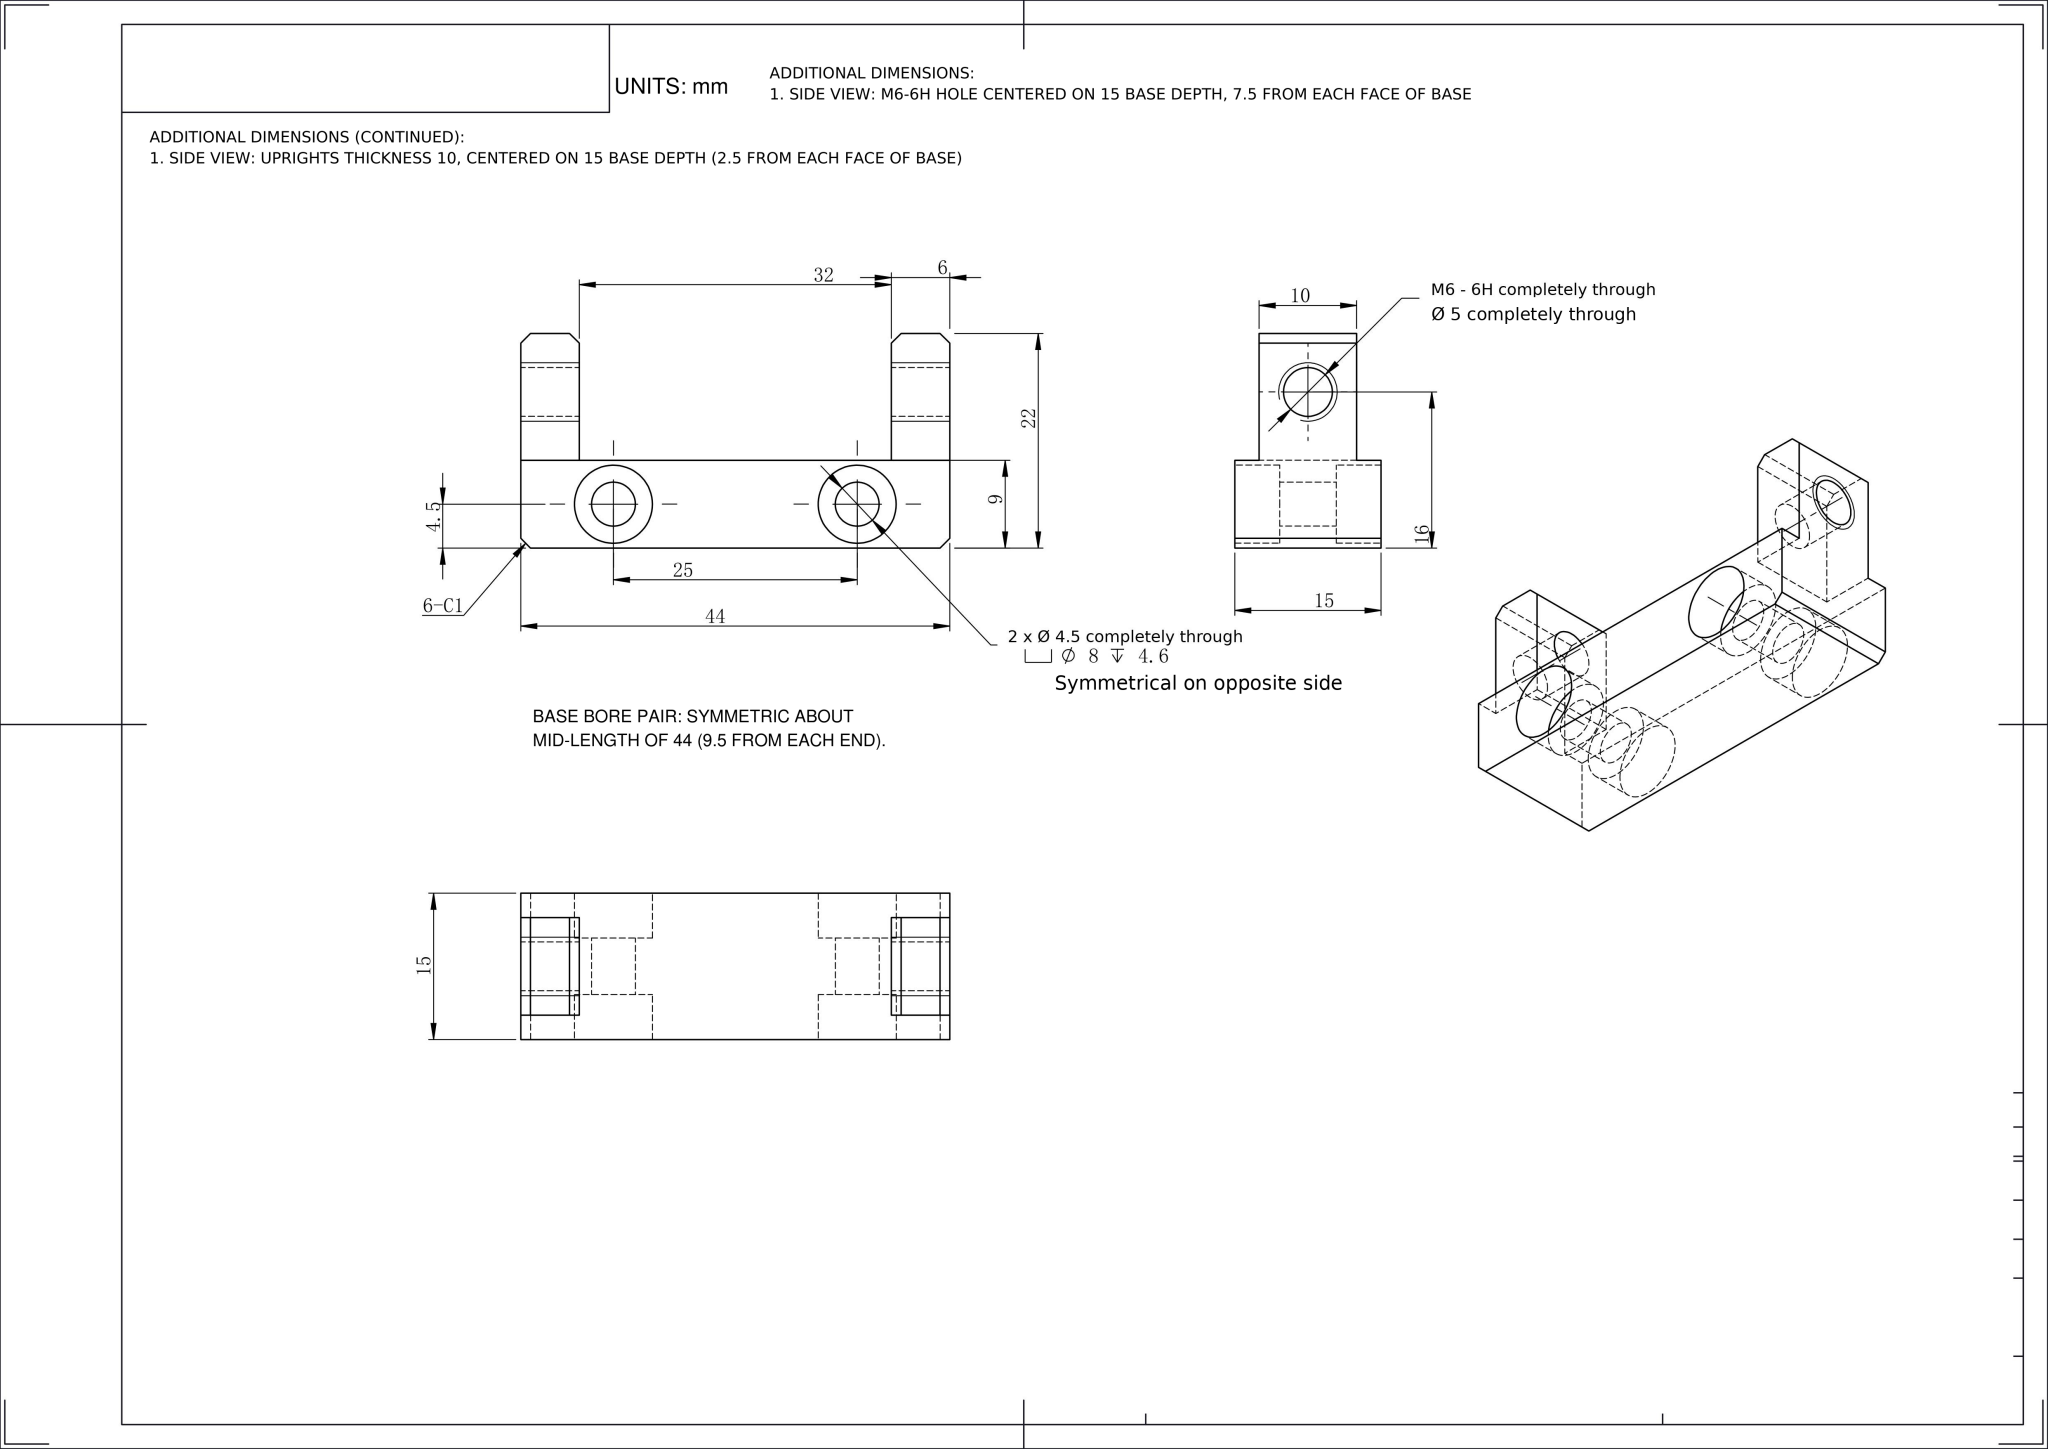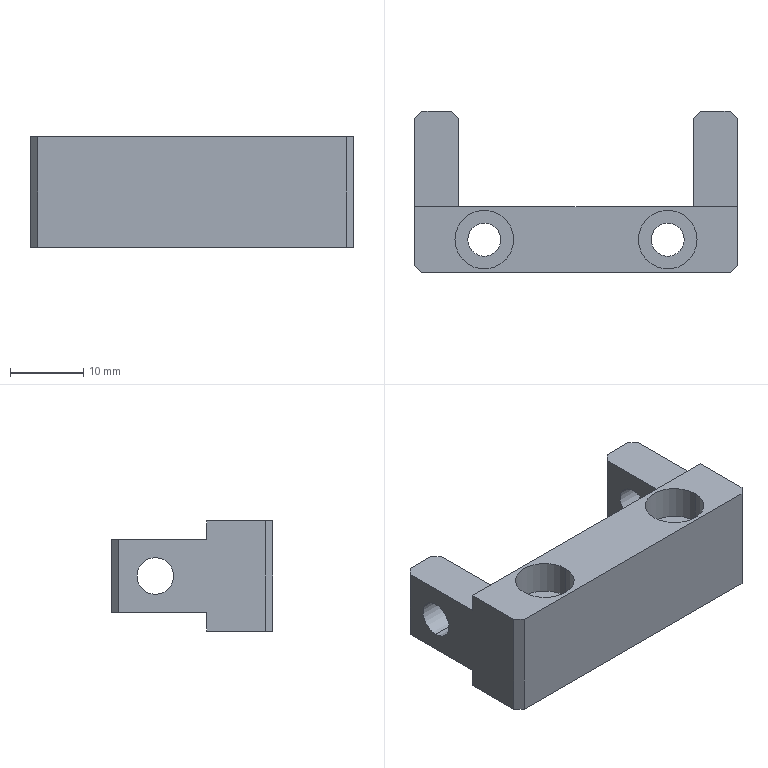Part | NX | mm | 1 solid | 40 faces | box 44 x 22 x 15 mm | volume 6120 mm3 | plane 24 | cylinder 16 | commonest cylinder face diameters 8 x8 4.5 x4 5 x4